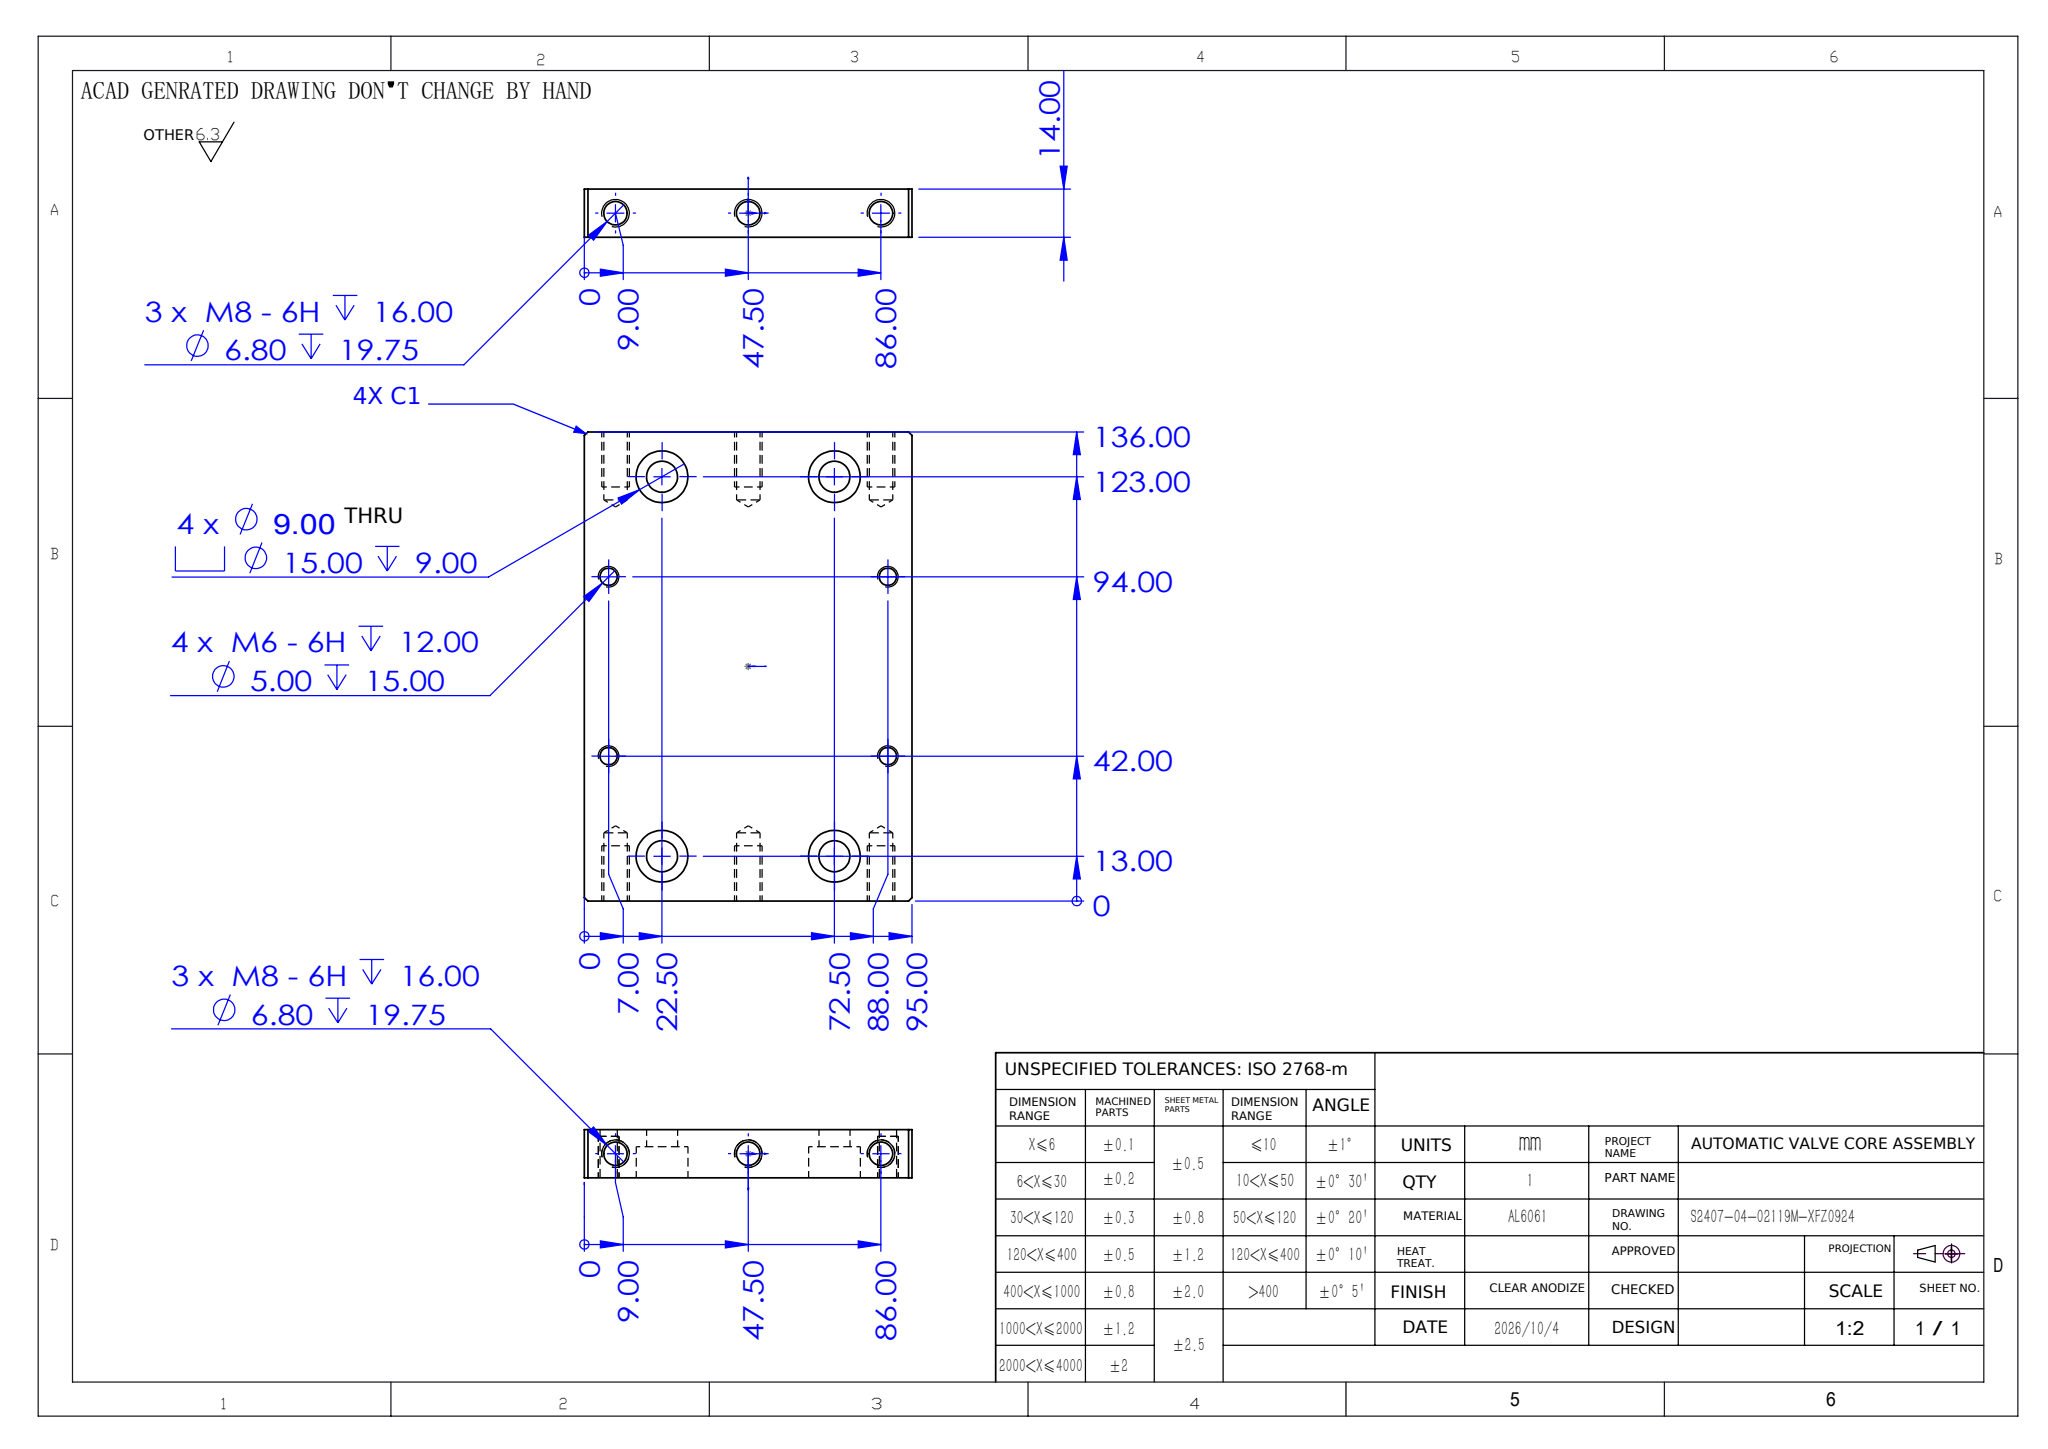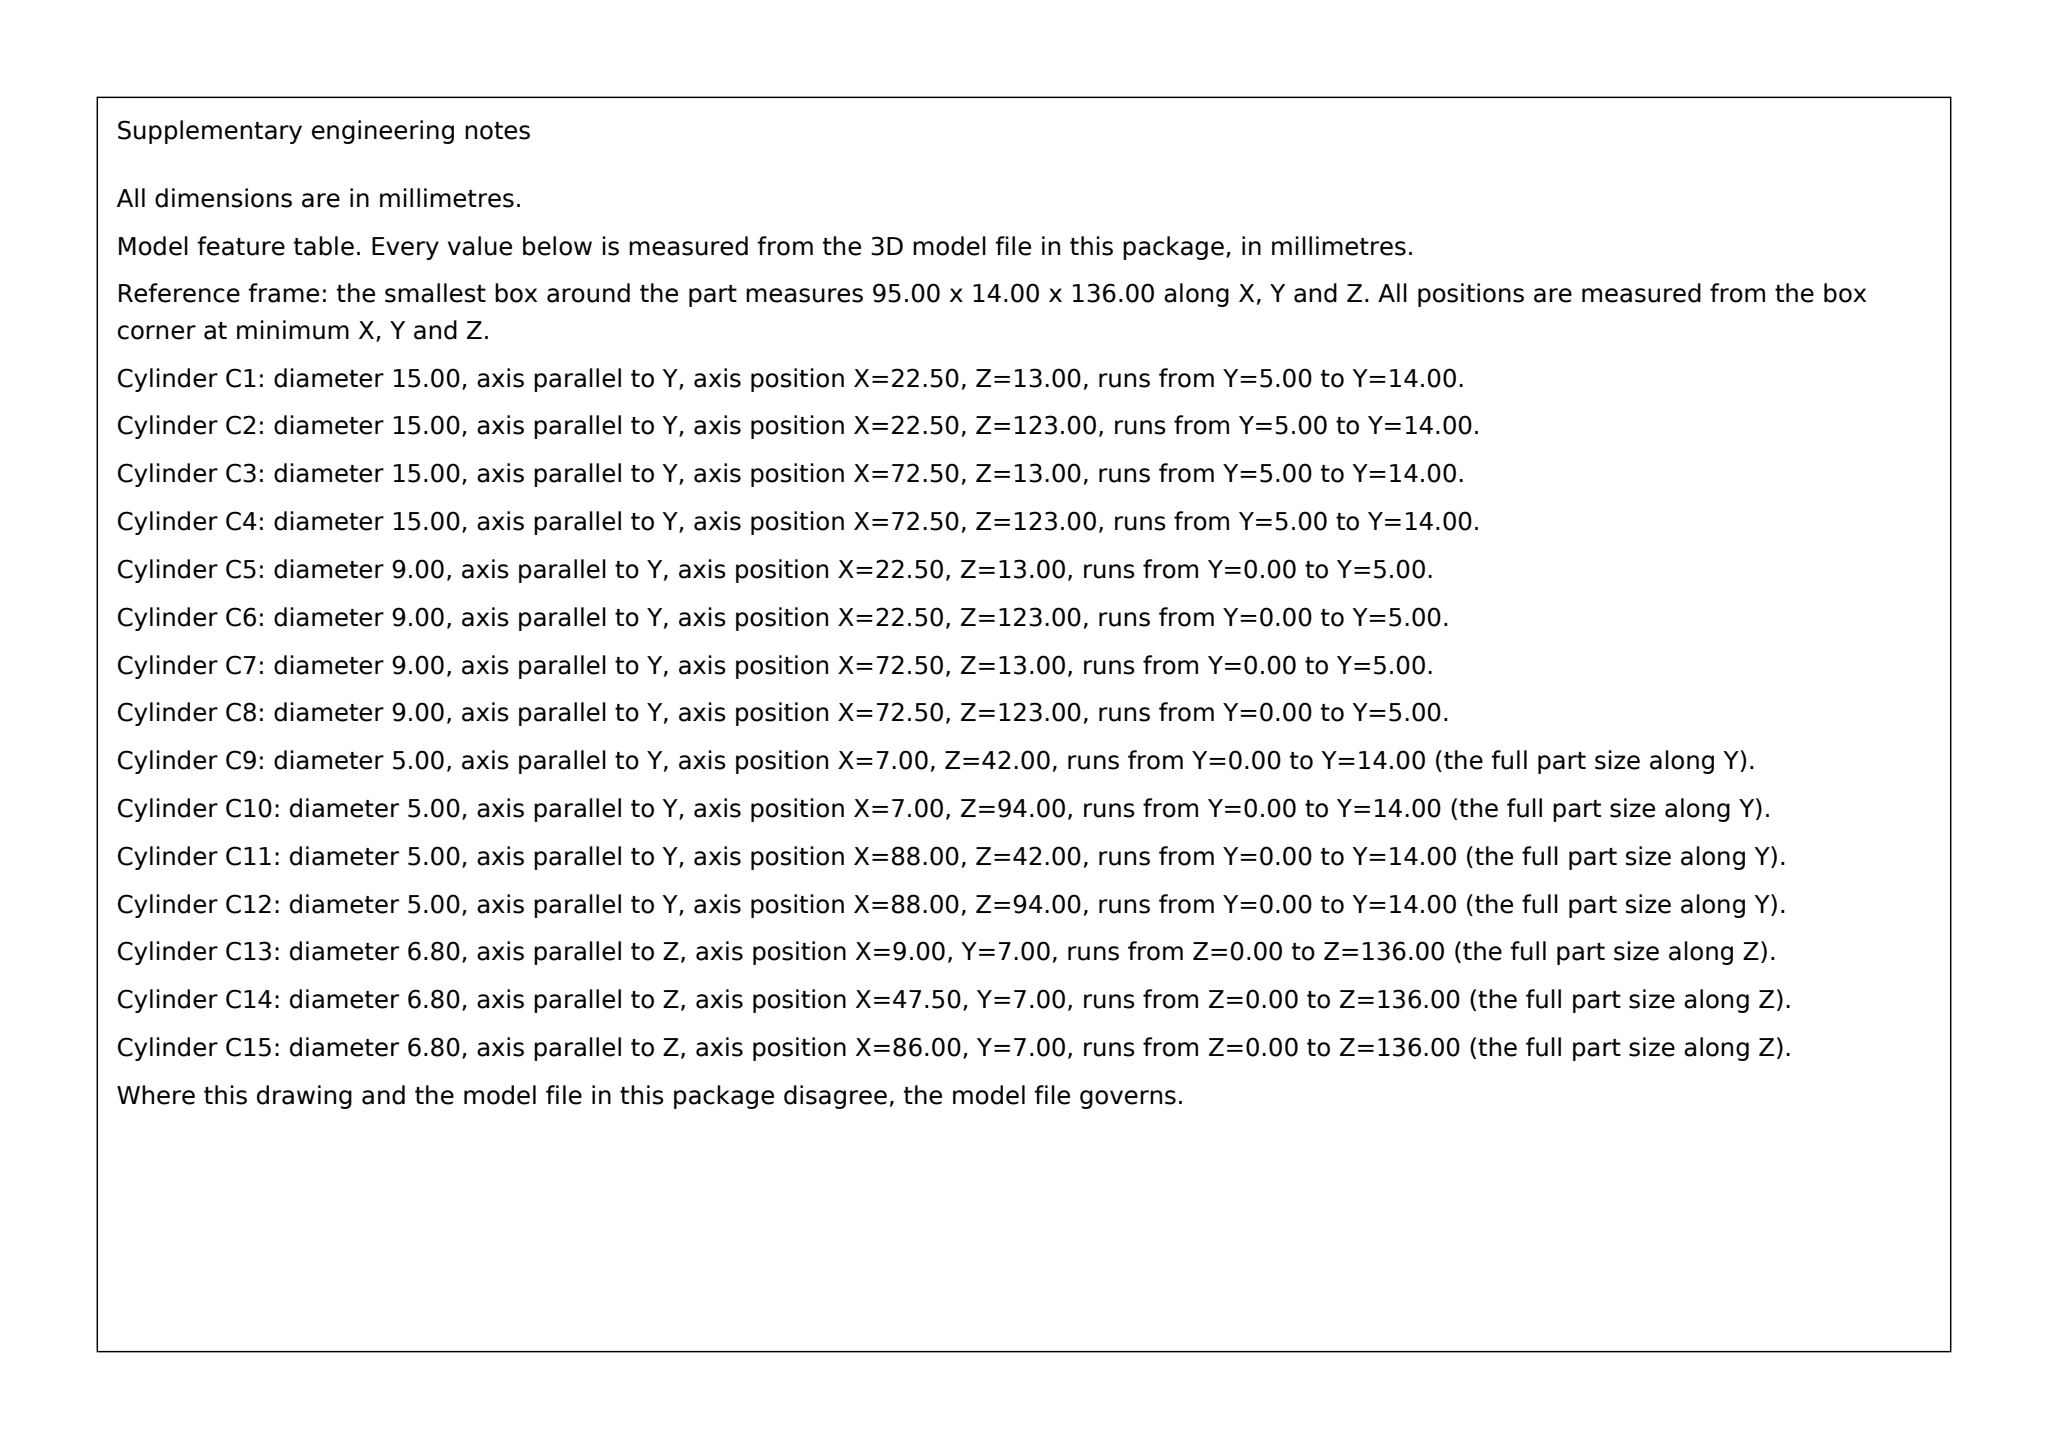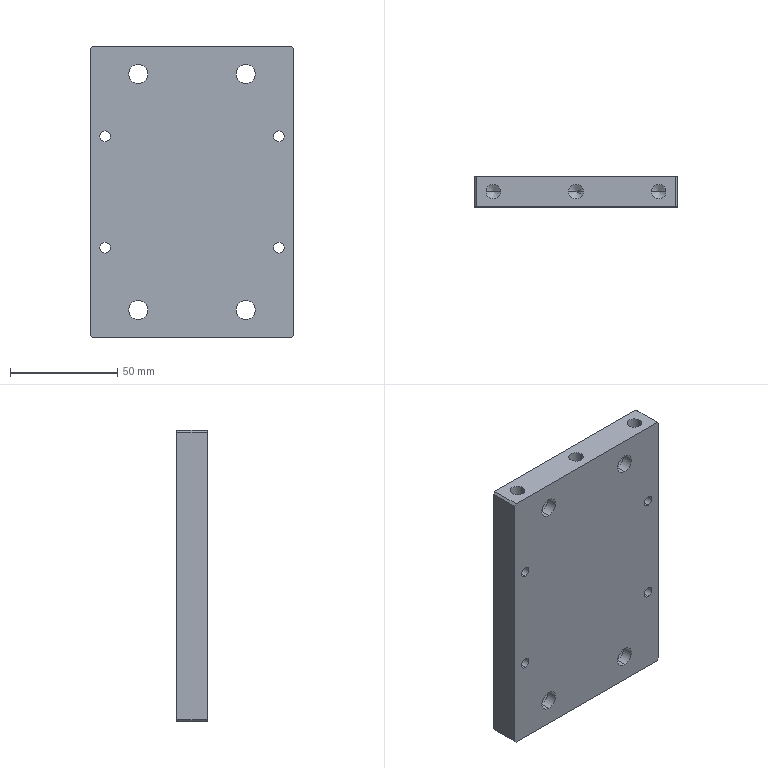Part | SolidWorks | mm | 1 solid | 62 faces | box 95 x 14 x 136 mm | volume 167666 mm3 | cylinder 36 | plane 14 | cone 12 | commonest cylinder face diameters 6.8 x12 5 x8 15 x8 9 x8
build123d program:
from build123d import *

# Parameters (mm, degrees)
SKETCH1_W                                         = 95
SKETCH1_H                                         = 136
BOSS_EXTRUDE1_DEPTH                               = 7
HOLE_SIZE_ACCORDING_TO_HEXAGON_SOCKET_D           = 9
HOLE_SIZE_ACCORDING_TO_HEXAGON_SOCKET_CBORE_D     = 15
HOLE_SIZE_ACCORDING_TO_HEXAGON_SOCKET_CBORE_DEPTH = 9
M8_TAPPED_HOLE1_D                                 = 6.8
M8_TAPPED_HOLE1_DEPTH                             = 19.75
M8_TAPPED_HOLE1_TIP                               = 2.043
M8_TAPPED_HOLE2_D                                 = 6.8
M8_TAPPED_HOLE2_DEPTH                             = 19.75
M8_TAPPED_HOLE2_TIP                               = 2.043
M6_TAPPED_HOLE1_D                                 = 5
M6_TAPPED_HOLE1_DEPTH                             = 15
M6_TAPPED_HOLE1_TIP                               = 1.502
CHAMFER1_SIZE                                     = 1


with BuildPart() as part:
    # Sketch1 → Boss-Extrude1 (new, symmetric)
    with BuildSketch(Plane(origin=(0, 0, 0), x_dir=(1, 0, 0), z_dir=(0, 1, 0))):
        Rectangle(SKETCH1_W, SKETCH1_H)
    extrude(amount=BOSS_EXTRUDE1_DEPTH, both=True)

    # Hole Size _According to_ Hexagon Socket (through all)
    with Locations(Plane(origin=(0, 7, 0), x_dir=(1, 0, 0), z_dir=(0, 1, 0))):
        with Locations((-25, -55), (-25, 55), (25, 55), (25, -55)):
            CounterBoreHole(HOLE_SIZE_ACCORDING_TO_HEXAGON_SOCKET_D / 2, HOLE_SIZE_ACCORDING_TO_HEXAGON_SOCKET_CBORE_D / 2, HOLE_SIZE_ACCORDING_TO_HEXAGON_SOCKET_CBORE_DEPTH)

    # M8 Tapped Hole1
    with Locations(Plane.XY.offset(68)):
        with Locations((0, 0), (-38.5, 0), (38.5, 0)):
            Hole(M8_TAPPED_HOLE1_D / 2, depth=M8_TAPPED_HOLE1_DEPTH)
            with Locations((0, 0, -(M8_TAPPED_HOLE1_DEPTH + M8_TAPPED_HOLE1_TIP / 2))):  # 118° drill point
                Cone(0, M8_TAPPED_HOLE1_D / 2, M8_TAPPED_HOLE1_TIP, mode=Mode.SUBTRACT)

    # M8 Tapped Hole2
    with Locations(Plane(origin=(0, 0, -68), x_dir=(-1, 0, 0), z_dir=(0, 0, -1))):
        with Locations((-38.5, 0), (0, 0), (38.5, 0)):
            Hole(M8_TAPPED_HOLE2_D / 2, depth=M8_TAPPED_HOLE2_DEPTH)
            with Locations((0, 0, -(M8_TAPPED_HOLE2_DEPTH + M8_TAPPED_HOLE2_TIP / 2))):  # 118° drill point
                Cone(0, M8_TAPPED_HOLE2_D / 2, M8_TAPPED_HOLE2_TIP, mode=Mode.SUBTRACT)

    # M6 Tapped Hole1
    with Locations(Plane(origin=(0, 7, 0), x_dir=(1, 0, 0), z_dir=(0, 1, 0))):
        with Locations((-40.5, -26), (-40.5, 26), (40.5, 26), (40.5, -26)):
            Hole(M6_TAPPED_HOLE1_D / 2, depth=M6_TAPPED_HOLE1_DEPTH)
            with Locations((0, 0, -(M6_TAPPED_HOLE1_DEPTH + M6_TAPPED_HOLE1_TIP / 2))):  # 118° drill point
                Cone(0, M6_TAPPED_HOLE1_D / 2, M6_TAPPED_HOLE1_TIP, mode=Mode.SUBTRACT)

    # Chamfer1
    chamfer1_edges = [part.edges().sort_by_distance(p)[0] for p in [
        (47.5, 0, 68),
        (-47.5, 0, 68),
        (-47.5, 0, -68),
        (47.5, 0, -68),
    ]]
    chamfer(chamfer1_edges, length=CHAMFER1_SIZE)


solid = part.part